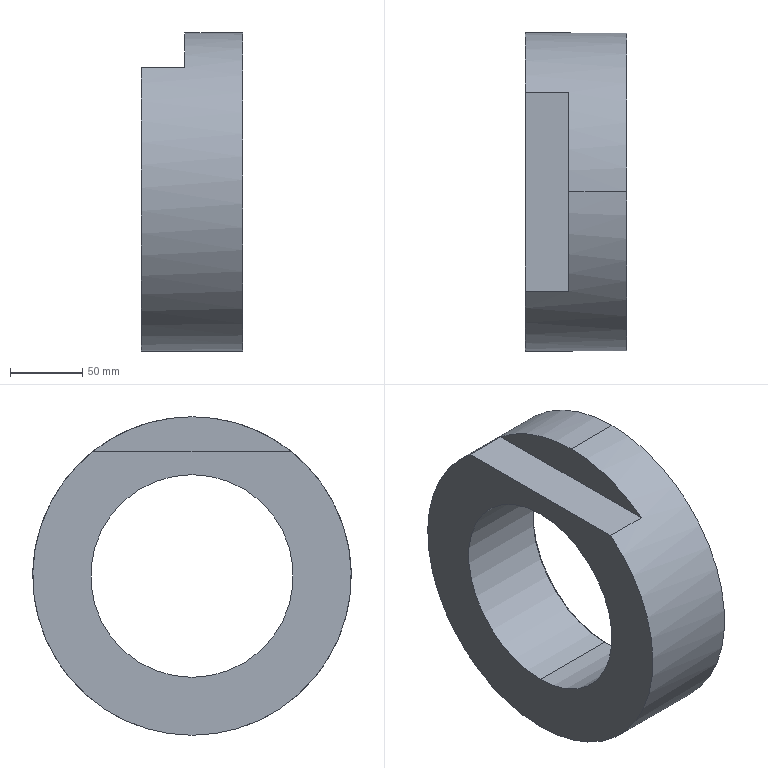Component | SolidWorks | JF21-80.1-1-3(_)-1-SOLID59-1 | 1 solid | 37 faces | box 70 x 220 x 220 mm | volume 1412143 mm3 | cylinder 18 | cone 14 | plane 5 | commonest cylinder face diameters 10.2 x12 205 x2 220 x2 140 x2
STEP:
#1=CARTESIAN_POINT('',(17.047,0.,24.37));
#2=VERTEX_POINT('',#1);
#3=CARTESIAN_POINT('',(17.047,0.,18.858));
#4=VERTEX_POINT('',#3);
#5=CARTESIAN_POINT('',(17.047,0.,21.614));
#6=DIRECTION('',(1.,0.,0.));
#7=DIRECTION('',(0.,0.,-1.));
#8=AXIS2_PLACEMENT_3D('',#5,#6,#7);
#9=CIRCLE('',#8,2.756);
#10=EDGE_CURVE('',#2,#4,#9,.T.);
#11=ORIENTED_EDGE('',*,*,#10,.F.);
#12=CARTESIAN_POINT('',(17.126,0.,24.449));
#13=VERTEX_POINT('',#12);
#14=CARTESIAN_POINT('',(17.126,0.,24.449));
#15=DIRECTION('',(-0.7071,-0.,-0.7071));
#16=VECTOR('',#15,39.37);
#17=LINE('',#14,#16);
#18=EDGE_CURVE('',#13,#2,#17,.T.);
#19=ORIENTED_EDGE('',*,*,#18,.F.);
#20=CARTESIAN_POINT('',(17.126,0.,18.78));
#21=VERTEX_POINT('',#20);
#22=CARTESIAN_POINT('',(17.126,0.,21.614));
#23=DIRECTION('',(-1.,0.,0.));
#24=DIRECTION('',(0.,0.,-1.));
#25=AXIS2_PLACEMENT_3D('',#22,#23,#24);
#26=CIRCLE('',#25,2.835);
#27=EDGE_CURVE('',#21,#13,#26,.T.);
#28=ORIENTED_EDGE('',*,*,#27,.F.);
#29=CARTESIAN_POINT('',(17.126,0.,18.78));
#30=DIRECTION('',(-0.7071,0.,0.7071));
#31=VECTOR('',#30,39.37);
#32=LINE('',#29,#31);
#33=EDGE_CURVE('',#21,#4,#32,.T.);
#34=ORIENTED_EDGE('',*,*,#33,.T.);
#35=EDGE_LOOP('',(#11,#19,#28,#34));
#36=FACE_OUTER_BOUND('',#35,.T.);
#37=CARTESIAN_POINT('',(17.126,0.,21.614));
#38=DIRECTION('',(1.,0.,0.));
#39=DIRECTION('',(0.,0.,1.));
#40=AXIS2_PLACEMENT_3D('',#37,#38,#39);
#41=CONICAL_SURFACE('',#40,2.835,0.7854);
#42=ADVANCED_FACE('',(#36),#41,.F.);
#43=CARTESIAN_POINT('',(15.974,2.898,20.142));
#44=VERTEX_POINT('',#43);
#45=CARTESIAN_POINT('',(15.974,2.898,19.74));
#46=VERTEX_POINT('',#45);
#47=CARTESIAN_POINT('',(15.974,2.898,19.941));
#48=DIRECTION('',(1.,0.,0.));
#49=DIRECTION('',(0.,0.,-1.));
#50=AXIS2_PLACEMENT_3D('',#47,#48,#49);
#51=CIRCLE('',#50,0.2008);
#52=EDGE_CURVE('',#44,#46,#51,.T.);
#53=ORIENTED_EDGE('',*,*,#52,.F.);
#54=CARTESIAN_POINT('',(17.126,2.898,20.142));
#55=VERTEX_POINT('',#54);
#56=CARTESIAN_POINT('',(17.126,2.898,20.142));
#57=DIRECTION('',(-1.,0.,0.));
#58=VECTOR('',#57,39.37);
#59=LINE('',#56,#58);
#60=EDGE_CURVE('',#55,#44,#59,.T.);
#61=ORIENTED_EDGE('',*,*,#60,.F.);
#62=CARTESIAN_POINT('',(17.126,2.898,19.74));
#63=VERTEX_POINT('',#62);
#64=CARTESIAN_POINT('',(17.126,2.898,19.941));
#65=DIRECTION('',(1.,0.,0.));
#66=DIRECTION('',(0.,0.,-1.));
#67=AXIS2_PLACEMENT_3D('',#64,#65,#66);
#68=CIRCLE('',#67,0.2008);
#69=EDGE_CURVE('',#55,#63,#68,.T.);
#70=ORIENTED_EDGE('',*,*,#69,.T.);
#71=CARTESIAN_POINT('',(17.126,2.898,19.74));
#72=DIRECTION('',(-1.,0.,0.));
#73=VECTOR('',#72,39.37);
#74=LINE('',#71,#73);
#75=EDGE_CURVE('',#63,#46,#74,.T.);
#76=ORIENTED_EDGE('',*,*,#75,.T.);
#77=EDGE_LOOP('',(#53,#61,#70,#76));
#78=FACE_OUTER_BOUND('',#77,.T.);
#79=CARTESIAN_POINT('',(17.126,2.898,19.941));
#80=DIRECTION('',(1.,0.,0.));
#81=DIRECTION('',(0.,0.,1.));
#82=AXIS2_PLACEMENT_3D('',#79,#80,#81);
#83=CYLINDRICAL_SURFACE('',#82,0.2008);
#84=ADVANCED_FACE('',(#78),#83,.F.);
#85=CARTESIAN_POINT('',(15.854,2.898,19.941));
#86=VERTEX_POINT('',#85);
#87=CARTESIAN_POINT('',(15.974,2.898,19.74));
#88=DIRECTION('',(-0.515,0.,0.8572));
#89=VECTOR('',#88,39.37);
#90=LINE('',#87,#89);
#91=EDGE_CURVE('',#46,#86,#90,.T.);
#92=ORIENTED_EDGE('',*,*,#91,.T.);
#93=CARTESIAN_POINT('',(15.974,2.898,20.142));
#94=DIRECTION('',(-0.515,-0.,-0.8572));
#95=VECTOR('',#94,39.37);
#96=LINE('',#93,#95);
#97=EDGE_CURVE('',#44,#86,#96,.T.);
#98=ORIENTED_EDGE('',*,*,#97,.F.);
#99=ORIENTED_EDGE('',*,*,#52,.T.);
#100=EDGE_LOOP('',(#92,#98,#99));
#101=FACE_OUTER_BOUND('',#100,.T.);
#102=CARTESIAN_POINT('',(15.974,2.898,19.941));
#103=DIRECTION('',(1.,0.,0.));
#104=DIRECTION('',(0.,0.,1.));
#105=AXIS2_PLACEMENT_3D('',#102,#103,#104);
#106=CONICAL_SURFACE('',#105,0.2008,1.03);
#107=ADVANCED_FACE('',(#101),#106,.F.);
#108=CARTESIAN_POINT('',(15.974,2.898,23.488));
#109=VERTEX_POINT('',#108);
#110=CARTESIAN_POINT('',(15.974,2.898,23.087));
#111=VERTEX_POINT('',#110);
#112=CARTESIAN_POINT('',(15.974,2.898,23.287));
#113=DIRECTION('',(1.,0.,0.));
#114=DIRECTION('',(0.,0.,-1.));
#115=AXIS2_PLACEMENT_3D('',#112,#113,#114);
#116=CIRCLE('',#115,0.2008);
#117=EDGE_CURVE('',#109,#111,#116,.T.);
#118=ORIENTED_EDGE('',*,*,#117,.F.);
#119=CARTESIAN_POINT('',(17.126,2.898,23.488));
#120=VERTEX_POINT('',#119);
#121=CARTESIAN_POINT('',(17.126,2.898,23.488));
#122=DIRECTION('',(-1.,0.,0.));
#123=VECTOR('',#122,39.37);
#124=LINE('',#121,#123);
#125=EDGE_CURVE('',#120,#109,#124,.T.);
#126=ORIENTED_EDGE('',*,*,#125,.F.);
#127=CARTESIAN_POINT('',(17.126,2.898,23.087));
#128=VERTEX_POINT('',#127);
#129=CARTESIAN_POINT('',(17.126,2.898,23.287));
#130=DIRECTION('',(1.,0.,0.));
#131=DIRECTION('',(0.,0.,-1.));
#132=AXIS2_PLACEMENT_3D('',#129,#130,#131);
#133=CIRCLE('',#132,0.2008);
#134=EDGE_CURVE('',#120,#128,#133,.T.);
#135=ORIENTED_EDGE('',*,*,#134,.T.);
#136=CARTESIAN_POINT('',(17.126,2.898,23.087));
#137=DIRECTION('',(-1.,0.,0.));
#138=VECTOR('',#137,39.37);
#139=LINE('',#136,#138);
#140=EDGE_CURVE('',#128,#111,#139,.T.);
#141=ORIENTED_EDGE('',*,*,#140,.T.);
#142=EDGE_LOOP('',(#118,#126,#135,#141));
#143=FACE_OUTER_BOUND('',#142,.T.);
#144=CARTESIAN_POINT('',(17.126,2.898,23.287));
#145=DIRECTION('',(1.,0.,0.));
#146=DIRECTION('',(0.,0.,1.));
#147=AXIS2_PLACEMENT_3D('',#144,#145,#146);
#148=CYLINDRICAL_SURFACE('',#147,0.2008);
#149=ADVANCED_FACE('',(#143),#148,.F.);
#150=CARTESIAN_POINT('',(15.854,2.898,23.287));
#151=VERTEX_POINT('',#150);
#152=CARTESIAN_POINT('',(15.974,2.898,23.087));
#153=DIRECTION('',(-0.515,0.,0.8572));
#154=VECTOR('',#153,39.37);
#155=LINE('',#152,#154);
#156=EDGE_CURVE('',#111,#151,#155,.T.);
#157=ORIENTED_EDGE('',*,*,#156,.T.);
#158=CARTESIAN_POINT('',(15.974,2.898,23.488));
#159=DIRECTION('',(-0.515,-0.,-0.8572));
#160=VECTOR('',#159,39.37);
#161=LINE('',#158,#160);
#162=EDGE_CURVE('',#109,#151,#161,.T.);
#163=ORIENTED_EDGE('',*,*,#162,.F.);
#164=ORIENTED_EDGE('',*,*,#117,.T.);
#165=EDGE_LOOP('',(#157,#163,#164));
#166=FACE_OUTER_BOUND('',#165,.T.);
#167=CARTESIAN_POINT('',(15.974,2.898,23.287));
#168=DIRECTION('',(1.,0.,0.));
#169=DIRECTION('',(0.,0.,1.));
#170=AXIS2_PLACEMENT_3D('',#167,#168,#169);
#171=CONICAL_SURFACE('',#170,0.2008,1.03);
#172=ADVANCED_FACE('',(#166),#171,.F.);
#173=CARTESIAN_POINT('',(15.974,0.,25.161));
#174=VERTEX_POINT('',#173);
#175=CARTESIAN_POINT('',(15.974,0.,24.76));
#176=VERTEX_POINT('',#175);
#177=CARTESIAN_POINT('',(15.974,0.,24.961));
#178=DIRECTION('',(1.,0.,0.));
#179=DIRECTION('',(0.,0.,-1.));
#180=AXIS2_PLACEMENT_3D('',#177,#178,#179);
#181=CIRCLE('',#180,0.2008);
#182=EDGE_CURVE('',#174,#176,#181,.T.);
#183=ORIENTED_EDGE('',*,*,#182,.F.);
#184=CARTESIAN_POINT('',(17.126,0.,25.161));
#185=VERTEX_POINT('',#184);
#186=CARTESIAN_POINT('',(17.126,0.,25.161));
#187=DIRECTION('',(-1.,0.,0.));
#188=VECTOR('',#187,39.37);
#189=LINE('',#186,#188);
#190=EDGE_CURVE('',#185,#174,#189,.T.);
#191=ORIENTED_EDGE('',*,*,#190,.F.);
#192=CARTESIAN_POINT('',(17.126,0.,24.76));
#193=VERTEX_POINT('',#192);
#194=CARTESIAN_POINT('',(17.126,0.,24.961));
#195=DIRECTION('',(1.,0.,0.));
#196=DIRECTION('',(0.,0.,-1.));
#197=AXIS2_PLACEMENT_3D('',#194,#195,#196);
#198=CIRCLE('',#197,0.2008);
#199=EDGE_CURVE('',#185,#193,#198,.T.);
#200=ORIENTED_EDGE('',*,*,#199,.T.);
#201=CARTESIAN_POINT('',(17.126,0.,24.76));
#202=DIRECTION('',(-1.,0.,0.));
#203=VECTOR('',#202,39.37);
#204=LINE('',#201,#203);
#205=EDGE_CURVE('',#193,#176,#204,.T.);
#206=ORIENTED_EDGE('',*,*,#205,.T.);
#207=EDGE_LOOP('',(#183,#191,#200,#206));
#208=FACE_OUTER_BOUND('',#207,.T.);
#209=CARTESIAN_POINT('',(17.126,0.,24.961));
#210=DIRECTION('',(1.,0.,0.));
#211=DIRECTION('',(0.,0.,1.));
#212=AXIS2_PLACEMENT_3D('',#209,#210,#211);
#213=CYLINDRICAL_SURFACE('',#212,0.2008);
#214=ADVANCED_FACE('',(#208),#213,.F.);
#215=CARTESIAN_POINT('',(15.854,0.,24.961));
#216=VERTEX_POINT('',#215);
#217=CARTESIAN_POINT('',(15.974,0.,24.76));
#218=DIRECTION('',(-0.515,0.,0.8572));
#219=VECTOR('',#218,39.37);
#220=LINE('',#217,#219);
#221=EDGE_CURVE('',#176,#216,#220,.T.);
#222=ORIENTED_EDGE('',*,*,#221,.T.);
#223=CARTESIAN_POINT('',(15.974,0.,25.161));
#224=DIRECTION('',(-0.515,-0.,-0.8572));
#225=VECTOR('',#224,39.37);
#226=LINE('',#223,#225);
#227=EDGE_CURVE('',#174,#216,#226,.T.);
#228=ORIENTED_EDGE('',*,*,#227,.F.);
#229=ORIENTED_EDGE('',*,*,#182,.T.);
#230=EDGE_LOOP('',(#222,#228,#229));
#231=FACE_OUTER_BOUND('',#230,.T.);
#232=CARTESIAN_POINT('',(15.974,0.,24.961));
#233=DIRECTION('',(1.,0.,0.));
#234=DIRECTION('',(0.,0.,1.));
#235=AXIS2_PLACEMENT_3D('',#232,#233,#234);
#236=CONICAL_SURFACE('',#235,0.2008,1.03);
#237=ADVANCED_FACE('',(#231),#236,.F.);
#238=CARTESIAN_POINT('',(15.974,-2.898,23.488));
#239=VERTEX_POINT('',#238);
#240=CARTESIAN_POINT('',(15.974,-2.898,23.087));
#241=VERTEX_POINT('',#240);
#242=CARTESIAN_POINT('',(15.974,-2.898,23.287));
#243=DIRECTION('',(1.,0.,0.));
#244=DIRECTION('',(0.,0.,-1.));
#245=AXIS2_PLACEMENT_3D('',#242,#243,#244);
#246=CIRCLE('',#245,0.2008);
#247=EDGE_CURVE('',#239,#241,#246,.T.);
#248=ORIENTED_EDGE('',*,*,#247,.F.);
#249=CARTESIAN_POINT('',(17.126,-2.898,23.488));
#250=VERTEX_POINT('',#249);
#251=CARTESIAN_POINT('',(17.126,-2.898,23.488));
#252=DIRECTION('',(-1.,0.,0.));
#253=VECTOR('',#252,39.37);
#254=LINE('',#251,#253);
#255=EDGE_CURVE('',#250,#239,#254,.T.);
#256=ORIENTED_EDGE('',*,*,#255,.F.);
#257=CARTESIAN_POINT('',(17.126,-2.898,23.087));
#258=VERTEX_POINT('',#257);
#259=CARTESIAN_POINT('',(17.126,-2.898,23.287));
#260=DIRECTION('',(1.,0.,0.));
#261=DIRECTION('',(0.,0.,-1.));
#262=AXIS2_PLACEMENT_3D('',#259,#260,#261);
#263=CIRCLE('',#262,0.2008);
#264=EDGE_CURVE('',#250,#258,#263,.T.);
#265=ORIENTED_EDGE('',*,*,#264,.T.);
#266=CARTESIAN_POINT('',(17.126,-2.898,23.087));
#267=DIRECTION('',(-1.,0.,0.));
#268=VECTOR('',#267,39.37);
#269=LINE('',#266,#268);
#270=EDGE_CURVE('',#258,#241,#269,.T.);
#271=ORIENTED_EDGE('',*,*,#270,.T.);
#272=EDGE_LOOP('',(#248,#256,#265,#271));
#273=FACE_OUTER_BOUND('',#272,.T.);
#274=CARTESIAN_POINT('',(17.126,-2.898,23.287));
#275=DIRECTION('',(1.,0.,0.));
#276=DIRECTION('',(0.,0.,1.));
#277=AXIS2_PLACEMENT_3D('',#274,#275,#276);
#278=CYLINDRICAL_SURFACE('',#277,0.2008);
#279=ADVANCED_FACE('',(#273),#278,.F.);
#280=CARTESIAN_POINT('',(15.854,-2.898,23.287));
#281=VERTEX_POINT('',#280);
#282=CARTESIAN_POINT('',(15.974,-2.898,23.087));
#283=DIRECTION('',(-0.515,0.,0.8572));
#284=VECTOR('',#283,39.37);
#285=LINE('',#282,#284);
#286=EDGE_CURVE('',#241,#281,#285,.T.);
#287=ORIENTED_EDGE('',*,*,#286,.T.);
#288=CARTESIAN_POINT('',(15.974,-2.898,23.488));
#289=DIRECTION('',(-0.515,-0.,-0.8572));
#290=VECTOR('',#289,39.37);
#291=LINE('',#288,#290);
#292=EDGE_CURVE('',#239,#281,#291,.T.);
#293=ORIENTED_EDGE('',*,*,#292,.F.);
#294=ORIENTED_EDGE('',*,*,#247,.T.);
#295=EDGE_LOOP('',(#287,#293,#294));
#296=FACE_OUTER_BOUND('',#295,.T.);
#297=CARTESIAN_POINT('',(15.974,-2.898,23.287));
#298=DIRECTION('',(1.,0.,0.));
#299=DIRECTION('',(0.,0.,1.));
#300=AXIS2_PLACEMENT_3D('',#297,#298,#299);
#301=CONICAL_SURFACE('',#300,0.2008,1.03);
#302=ADVANCED_FACE('',(#296),#301,.F.);
#303=CARTESIAN_POINT('',(15.974,-2.898,20.142));
#304=VERTEX_POINT('',#303);
#305=CARTESIAN_POINT('',(15.974,-2.898,19.74));
#306=VERTEX_POINT('',#305);
#307=CARTESIAN_POINT('',(15.974,-2.898,19.941));
#308=DIRECTION('',(1.,0.,0.));
#309=DIRECTION('',(0.,0.,-1.));
#310=AXIS2_PLACEMENT_3D('',#307,#308,#309);
#311=CIRCLE('',#310,0.2008);
#312=EDGE_CURVE('',#304,#306,#311,.T.);
#313=ORIENTED_EDGE('',*,*,#312,.F.);
#314=CARTESIAN_POINT('',(17.126,-2.898,20.142));
#315=VERTEX_POINT('',#314);
#316=CARTESIAN_POINT('',(17.126,-2.898,20.142));
#317=DIRECTION('',(-1.,0.,0.));
#318=VECTOR('',#317,39.37);
#319=LINE('',#316,#318);
#320=EDGE_CURVE('',#315,#304,#319,.T.);
#321=ORIENTED_EDGE('',*,*,#320,.F.);
#322=CARTESIAN_POINT('',(17.126,-2.898,19.74));
#323=VERTEX_POINT('',#322);
#324=CARTESIAN_POINT('',(17.126,-2.898,19.941));
#325=DIRECTION('',(1.,0.,0.));
#326=DIRECTION('',(0.,0.,-1.));
#327=AXIS2_PLACEMENT_3D('',#324,#325,#326);
#328=CIRCLE('',#327,0.2008);
#329=EDGE_CURVE('',#315,#323,#328,.T.);
#330=ORIENTED_EDGE('',*,*,#329,.T.);
#331=CARTESIAN_POINT('',(17.126,-2.898,19.74));
#332=DIRECTION('',(-1.,0.,0.));
#333=VECTOR('',#332,39.37);
#334=LINE('',#331,#333);
#335=EDGE_CURVE('',#323,#306,#334,.T.);
#336=ORIENTED_EDGE('',*,*,#335,.T.);
#337=EDGE_LOOP('',(#313,#321,#330,#336));
#338=FACE_OUTER_BOUND('',#337,.T.);
#339=CARTESIAN_POINT('',(17.126,-2.898,19.941));
#340=DIRECTION('',(1.,0.,0.));
#341=DIRECTION('',(0.,0.,1.));
#342=AXIS2_PLACEMENT_3D('',#339,#340,#341);
#343=CYLINDRICAL_SURFACE('',#342,0.2008);
#344=ADVANCED_FACE('',(#338),#343,.F.);
#345=CARTESIAN_POINT('',(15.854,-2.898,19.941));
#346=VERTEX_POINT('',#345);
#347=CARTESIAN_POINT('',(15.974,-2.898,19.74));
#348=DIRECTION('',(-0.515,0.,0.8572));
#349=VECTOR('',#348,39.37);
#350=LINE('',#347,#349);
#351=EDGE_CURVE('',#306,#346,#350,.T.);
#352=ORIENTED_EDGE('',*,*,#351,.T.);
#353=CARTESIAN_POINT('',(15.974,-2.898,20.142));
#354=DIRECTION('',(-0.515,-0.,-0.8572));
#355=VECTOR('',#354,39.37);
#356=LINE('',#353,#355);
#357=EDGE_CURVE('',#304,#346,#356,.T.);
#358=ORIENTED_EDGE('',*,*,#357,.F.);
#359=ORIENTED_EDGE('',*,*,#312,.T.);
#360=EDGE_LOOP('',(#352,#358,#359));
#361=FACE_OUTER_BOUND('',#360,.T.);
#362=CARTESIAN_POINT('',(15.974,-2.898,19.941));
#363=DIRECTION('',(1.,0.,0.));
#364=DIRECTION('',(0.,0.,1.));
#365=AXIS2_PLACEMENT_3D('',#362,#363,#364);
#366=CONICAL_SURFACE('',#365,0.2008,1.03);
#367=ADVANCED_FACE('',(#361),#366,.F.);
#368=CARTESIAN_POINT('',(15.974,0.,18.469));
#369=VERTEX_POINT('',#368);
#370=CARTESIAN_POINT('',(15.974,0.,18.067));
#371=VERTEX_POINT('',#370);
#372=CARTESIAN_POINT('',(15.974,0.,18.268));
#373=DIRECTION('',(1.,0.,0.));
#374=DIRECTION('',(0.,0.,-1.));
#375=AXIS2_PLACEMENT_3D('',#372,#373,#374);
#376=CIRCLE('',#375,0.2008);
#377=EDGE_CURVE('',#369,#371,#376,.T.);
#378=ORIENTED_EDGE('',*,*,#377,.F.);
#379=CARTESIAN_POINT('',(17.126,0.,18.469));
#380=VERTEX_POINT('',#379);
#381=CARTESIAN_POINT('',(17.126,0.,18.469));
#382=DIRECTION('',(-1.,0.,0.));
#383=VECTOR('',#382,39.37);
#384=LINE('',#381,#383);
#385=EDGE_CURVE('',#380,#369,#384,.T.);
#386=ORIENTED_EDGE('',*,*,#385,.F.);
#387=CARTESIAN_POINT('',(17.126,0.,18.067));
#388=VERTEX_POINT('',#387);
#389=CARTESIAN_POINT('',(17.126,0.,18.268));
#390=DIRECTION('',(1.,0.,0.));
#391=DIRECTION('',(0.,0.,-1.));
#392=AXIS2_PLACEMENT_3D('',#389,#390,#391);
#393=CIRCLE('',#392,0.2008);
#394=EDGE_CURVE('',#380,#388,#393,.T.);
#395=ORIENTED_EDGE('',*,*,#394,.T.);
#396=CARTESIAN_POINT('',(17.126,0.,18.067));
#397=DIRECTION('',(-1.,0.,0.));
#398=VECTOR('',#397,39.37);
#399=LINE('',#396,#398);
#400=EDGE_CURVE('',#388,#371,#399,.T.);
#401=ORIENTED_EDGE('',*,*,#400,.T.);
#402=EDGE_LOOP('',(#378,#386,#395,#401));
#403=FACE_OUTER_BOUND('',#402,.T.);
#404=CARTESIAN_POINT('',(17.126,0.,18.268));
#405=DIRECTION('',(1.,0.,0.));
#406=DIRECTION('',(0.,0.,1.));
#407=AXIS2_PLACEMENT_3D('',#404,#405,#406);
#408=CYLINDRICAL_SURFACE('',#407,0.2008);
#409=ADVANCED_FACE('',(#403),#408,.F.);
#410=CARTESIAN_POINT('',(15.854,-0.,18.268));
#411=VERTEX_POINT('',#410);
#412=CARTESIAN_POINT('',(15.974,0.,18.067));
#413=DIRECTION('',(-0.515,0.,0.8572));
#414=VECTOR('',#413,39.37);
#415=LINE('',#412,#414);
#416=EDGE_CURVE('',#371,#411,#415,.T.);
#417=ORIENTED_EDGE('',*,*,#416,.T.);
#418=CARTESIAN_POINT('',(15.974,0.,18.469));
#419=DIRECTION('',(-0.515,-0.,-0.8572));
#420=VECTOR('',#419,39.37);
#421=LINE('',#418,#420);
#422=EDGE_CURVE('',#369,#411,#421,.T.);
#423=ORIENTED_EDGE('',*,*,#422,.F.);
#424=ORIENTED_EDGE('',*,*,#377,.T.);
#425=EDGE_LOOP('',(#417,#423,#424));
#426=FACE_OUTER_BOUND('',#425,.T.);
#427=CARTESIAN_POINT('',(15.974,0.,18.268));
#428=DIRECTION('',(1.,0.,0.));
#429=DIRECTION('',(0.,0.,1.));
#430=AXIS2_PLACEMENT_3D('',#427,#428,#429);
#431=CONICAL_SURFACE('',#430,0.2008,1.03);
#432=ADVANCED_FACE('',(#426),#431,.F.);
#433=CARTESIAN_POINT('',(17.126,0.,25.65));
#434=VERTEX_POINT('',#433);
#435=CARTESIAN_POINT('',(17.126,0.,17.579));
#436=VERTEX_POINT('',#435);
#437=CARTESIAN_POINT('',(17.126,0.,21.614));
#438=DIRECTION('',(1.,0.,0.));
#439=DIRECTION('',(0.,0.,-1.));
#440=AXIS2_PLACEMENT_3D('',#437,#438,#439);
#441=CIRCLE('',#440,4.035);
#442=EDGE_CURVE('',#434,#436,#441,.T.);
#443=ORIENTED_EDGE('',*,*,#442,.F.);
#444=CARTESIAN_POINT('',(17.323,0.,25.65));
#445=VERTEX_POINT('',#444);
#446=CARTESIAN_POINT('',(17.126,0.,25.65));
#447=DIRECTION('',(-1.,0.,0.));
#448=VECTOR('',#447,39.37);
#449=LINE('',#446,#448);
#450=EDGE_CURVE('',#445,#434,#449,.T.);
#451=ORIENTED_EDGE('',*,*,#450,.F.);
#452=CARTESIAN_POINT('',(17.323,0.,17.579));
#453=VERTEX_POINT('',#452);
#454=CARTESIAN_POINT('',(17.323,0.,21.614));
#455=DIRECTION('',(1.,0.,0.));
#456=DIRECTION('',(0.,0.,-1.));
#457=AXIS2_PLACEMENT_3D('',#454,#455,#456);
#458=CIRCLE('',#457,4.035);
#459=EDGE_CURVE('',#445,#453,#458,.T.);
#460=ORIENTED_EDGE('',*,*,#459,.T.);
#461=CARTESIAN_POINT('',(17.126,0.,17.579));
#462=DIRECTION('',(-1.,0.,0.));
#463=VECTOR('',#462,39.37);
#464=LINE('',#461,#463);
#465=EDGE_CURVE('',#453,#436,#464,.T.);
#466=ORIENTED_EDGE('',*,*,#465,.T.);
#467=EDGE_LOOP('',(#443,#451,#460,#466));
#468=FACE_OUTER_BOUND('',#467,.T.);
#469=CARTESIAN_POINT('',(17.126,0.,21.614));
#470=DIRECTION('',(1.,0.,0.));
#471=DIRECTION('',(0.,0.,1.));
#472=AXIS2_PLACEMENT_3D('',#469,#470,#471);
#473=CYLINDRICAL_SURFACE('',#472,4.035);
#474=ADVANCED_FACE('',(#468),#473,.F.);
#475=CARTESIAN_POINT('',(15.748,0.,25.945));
#476=VERTEX_POINT('',#475);
#477=CARTESIAN_POINT('',(15.748,2.7,25.));
#478=VERTEX_POINT('',#477);
#479=CARTESIAN_POINT('',(15.748,0.,21.614));
#480=DIRECTION('',(-1.,0.,0.));
#481=DIRECTION('',(0.,0.,1.));
#482=AXIS2_PLACEMENT_3D('',#479,#480,#481);
#483=CIRCLE('',#482,4.331);
#484=EDGE_CURVE('',#476,#478,#483,.T.);
#485=ORIENTED_EDGE('',*,*,#484,.F.);
#486=CARTESIAN_POINT('',(17.323,0.,25.945));
#487=VERTEX_POINT('',#486);
#488=CARTESIAN_POINT('',(14.567,0.,25.945));
#489=DIRECTION('',(-1.,0.,0.));
#490=VECTOR('',#489,39.37);
#491=LINE('',#488,#490);
#492=EDGE_CURVE('',#487,#476,#491,.T.);
#493=ORIENTED_EDGE('',*,*,#492,.F.);
#494=CARTESIAN_POINT('',(17.323,0.,17.283));
#495=VERTEX_POINT('',#494);
#496=CARTESIAN_POINT('',(17.323,0.,21.614));
#497=DIRECTION('',(1.,0.,0.));
#498=DIRECTION('',(0.,0.,-1.));
#499=AXIS2_PLACEMENT_3D('',#496,#497,#498);
#500=CIRCLE('',#499,4.331);
#501=EDGE_CURVE('',#495,#487,#500,.T.);
#502=ORIENTED_EDGE('',*,*,#501,.F.);
#503=CARTESIAN_POINT('',(14.567,0.,17.283));
#504=VERTEX_POINT('',#503);
#505=CARTESIAN_POINT('',(14.567,0.,17.283));
#506=DIRECTION('',(-1.,0.,0.));
#507=VECTOR('',#506,39.37);
#508=LINE('',#505,#507);
#509=EDGE_CURVE('',#495,#504,#508,.T.);
#510=ORIENTED_EDGE('',*,*,#509,.T.);
#511=CARTESIAN_POINT('',(14.567,2.7,25.));
#512=VERTEX_POINT('',#511);
#513=CARTESIAN_POINT('',(14.567,0.,21.614));
#514=DIRECTION('',(1.,0.,0.));
#515=DIRECTION('',(0.,0.,-1.));
#516=AXIS2_PLACEMENT_3D('',#513,#514,#515);
#517=CIRCLE('',#516,4.331);
#518=EDGE_CURVE('',#504,#512,#517,.T.);
#519=ORIENTED_EDGE('',*,*,#518,.T.);
#520=CARTESIAN_POINT('',(15.748,2.7,25.));
#521=DIRECTION('',(-1.,0.,0.));
#522=VECTOR('',#521,39.37);
#523=LINE('',#520,#522);
#524=EDGE_CURVE('',#478,#512,#523,.T.);
#525=ORIENTED_EDGE('',*,*,#524,.F.);
#526=EDGE_LOOP('',(#485,#493,#502,#510,#519,#525));
#527=FACE_OUTER_BOUND('',#526,.T.);
#528=CARTESIAN_POINT('',(14.567,0.,21.614));
#529=DIRECTION('',(1.,0.,0.));
#530=DIRECTION('',(0.,0.,1.));
#531=AXIS2_PLACEMENT_3D('',#528,#529,#530);
#532=CYLINDRICAL_SURFACE('',#531,4.331);
#533=ADVANCED_FACE('',(#527),#532,.T.);
#534=CARTESIAN_POINT('',(14.567,0.,24.37));
#535=VERTEX_POINT('',#534);
#536=CARTESIAN_POINT('',(14.567,0.,18.858));
#537=VERTEX_POINT('',#536);
#538=CARTESIAN_POINT('',(14.567,0.,21.614));
#539=DIRECTION('',(1.,0.,0.));
#540=DIRECTION('',(0.,0.,-1.));
#541=AXIS2_PLACEMENT_3D('',#538,#539,#540);
#542=CIRCLE('',#541,2.756);
#543=EDGE_CURVE('',#535,#537,#542,.T.);
#544=ORIENTED_EDGE('',*,*,#543,.F.);
#545=CARTESIAN_POINT('',(14.567,0.,24.37));
#546=DIRECTION('',(-1.,0.,0.));
#547=VECTOR('',#546,39.37);
#548=LINE('',#545,#547);
#549=EDGE_CURVE('',#2,#535,#548,.T.);
#550=ORIENTED_EDGE('',*,*,#549,.F.);
#551=ORIENTED_EDGE('',*,*,#10,.T.);
#552=CARTESIAN_POINT('',(14.567,0.,18.858));
#553=DIRECTION('',(-1.,0.,0.));
#554=VECTOR('',#553,39.37);
#555=LINE('',#552,#554);
#556=EDGE_CURVE('',#4,#537,#555,.T.);
#557=ORIENTED_EDGE('',*,*,#556,.T.);
#558=EDGE_LOOP('',(#544,#550,#551,#557));
#559=FACE_OUTER_BOUND('',#558,.T.);
#560=CARTESIAN_POINT('',(14.567,0.,21.614));
#561=DIRECTION('',(1.,0.,0.));
#562=DIRECTION('',(0.,0.,1.));
#563=AXIS2_PLACEMENT_3D('',#560,#561,#562);
#564=CYLINDRICAL_SURFACE('',#563,2.756);
#565=ADVANCED_FACE('',(#559),#564,.F.);
#566=ORIENTED_EDGE('',*,*,#549,.T.);
#567=CARTESIAN_POINT('',(14.567,0.,21.614));
#568=DIRECTION('',(1.,0.,0.));
#569=DIRECTION('',(0.,0.,-1.));
#570=AXIS2_PLACEMENT_3D('',#567,#568,#569);
#571=CIRCLE('',#570,2.756);
#572=EDGE_CURVE('',#537,#535,#571,.T.);
#573=ORIENTED_EDGE('',*,*,#572,.F.);
#574=ORIENTED_EDGE('',*,*,#556,.F.);
#575=CARTESIAN_POINT('',(17.047,0.,21.614));
#576=DIRECTION('',(1.,0.,0.));
#577=DIRECTION('',(0.,0.,-1.));
#578=AXIS2_PLACEMENT_3D('',#575,#576,#577);
#579=CIRCLE('',#578,2.756);
#580=EDGE_CURVE('',#4,#2,#579,.T.);
#581=ORIENTED_EDGE('',*,*,#580,.T.);
#582=EDGE_LOOP('',(#566,#573,#574,#581));
#583=FACE_OUTER_BOUND('',#582,.T.);
#584=CARTESIAN_POINT('',(14.567,0.,21.614));
#585=DIRECTION('',(1.,0.,0.));
#586=DIRECTION('',(0.,0.,1.));
#587=AXIS2_PLACEMENT_3D('',#584,#585,#586);
#588=CYLINDRICAL_SURFACE('',#587,2.756);
#589=ADVANCED_FACE('',(#583),#588,.F.);
#590=ORIENTED_EDGE('',*,*,#492,.T.);
#591=CARTESIAN_POINT('',(15.748,-2.7,25.));
#592=VERTEX_POINT('',#591);
#593=CARTESIAN_POINT('',(15.748,0.,21.614));
#594=DIRECTION('',(-1.,0.,0.));
#595=DIRECTION('',(0.,0.,1.));
#596=AXIS2_PLACEMENT_3D('',#593,#594,#595);
#597=CIRCLE('',#596,4.331);
#598=EDGE_CURVE('',#592,#476,#597,.T.);
#599=ORIENTED_EDGE('',*,*,#598,.F.);
#600=CARTESIAN_POINT('',(14.567,-2.7,25.));
#601=VERTEX_POINT('',#600);
#602=CARTESIAN_POINT('',(15.748,-2.7,25.));
#603=DIRECTION('',(-1.,0.,0.));
#604=VECTOR('',#603,39.37);
#605=LINE('',#602,#604);
#606=EDGE_CURVE('',#592,#601,#605,.T.);
#607=ORIENTED_EDGE('',*,*,#606,.T.);
#608=CARTESIAN_POINT('',(14.567,0.,21.614));
#609=DIRECTION('',(1.,0.,0.));
#610=DIRECTION('',(0.,0.,-1.));
#611=AXIS2_PLACEMENT_3D('',#608,#609,#610);
#612=CIRCLE('',#611,4.331);
#613=EDGE_CURVE('',#601,#504,#612,.T.);
#614=ORIENTED_EDGE('',*,*,#613,.T.);
#615=ORIENTED_EDGE('',*,*,#509,.F.);
#616=CARTESIAN_POINT('',(17.323,0.,21.614));
#617=DIRECTION('',(1.,0.,0.));
#618=DIRECTION('',(0.,0.,-1.));
#619=AXIS2_PLACEMENT_3D('',#616,#617,#618);
#620=CIRCLE('',#619,4.331);
#621=EDGE_CURVE('',#487,#495,#620,.T.);
#622=ORIENTED_EDGE('',*,*,#621,.F.);
#623=EDGE_LOOP('',(#590,#599,#607,#614,#615,#622));
#624=FACE_OUTER_BOUND('',#623,.T.);
#625=CARTESIAN_POINT('',(14.567,0.,21.614));
#626=DIRECTION('',(1.,0.,0.));
#627=DIRECTION('',(0.,0.,1.));
#628=AXIS2_PLACEMENT_3D('',#625,#626,#627);
#629=CYLINDRICAL_SURFACE('',#628,4.331);
#630=ADVANCED_FACE('',(#624),#629,.T.);
#631=ORIENTED_EDGE('',*,*,#572,.T.);
#632=ORIENTED_EDGE('',*,*,#543,.T.);
#633=EDGE_LOOP('',(#631,#632));
#634=FACE_BOUND('',#633,.T.);
#635=ORIENTED_EDGE('',*,*,#613,.F.);
#636=CARTESIAN_POINT('',(14.567,2.7,25.));
#637=DIRECTION('',(0.,-1.,0.));
#638=VECTOR('',#637,39.37);
#639=LINE('',#636,#638);
#640=EDGE_CURVE('',#512,#601,#639,.T.);
#641=ORIENTED_EDGE('',*,*,#640,.F.);
#642=ORIENTED_EDGE('',*,*,#518,.F.);
#643=EDGE_LOOP('',(#635,#641,#642));
#644=FACE_OUTER_BOUND('',#643,.T.);
#645=CARTESIAN_POINT('',(14.567,0.,21.614));
#646=DIRECTION('',(1.,0.,0.));
#647=DIRECTION('',(0.,0.,1.));
#648=AXIS2_PLACEMENT_3D('',#645,#646,#647);
#649=PLANE('',#648);
#650=ADVANCED_FACE('',(#634,#644),#649,.F.);
#651=CARTESIAN_POINT('',(17.323,0.,21.614));
#652=DIRECTION('',(1.,0.,0.));
#653=DIRECTION('',(0.,0.,-1.));
#654=AXIS2_PLACEMENT_3D('',#651,#652,#653);
#655=CIRCLE('',#654,4.035);
#656=EDGE_CURVE('',#453,#445,#655,.T.);
#657=ORIENTED_EDGE('',*,*,#656,.F.);
#658=ORIENTED_EDGE('',*,*,#459,.F.);
#659=EDGE_LOOP('',(#657,#658));
#660=FACE_BOUND('',#659,.T.);
#661=ORIENTED_EDGE('',*,*,#501,.T.);
#662=ORIENTED_EDGE('',*,*,#621,.T.);
#663=EDGE_LOOP('',(#661,#662));
#664=FACE_OUTER_BOUND('',#663,.T.);
#665=CARTESIAN_POINT('',(17.323,0.,21.614));
#666=DIRECTION('',(1.,0.,0.));
#667=DIRECTION('',(0.,0.,1.));
#668=AXIS2_PLACEMENT_3D('',#665,#666,#667);
#669=PLANE('',#668);
#670=ADVANCED_FACE('',(#660,#664),#669,.T.);
#671=ORIENTED_EDGE('',*,*,#640,.T.);
#672=ORIENTED_EDGE('',*,*,#606,.F.);
#673=CARTESIAN_POINT('',(15.748,2.7,25.));
#674=DIRECTION('',(0.,-1.,0.));
#675=VECTOR('',#674,39.37);
#676=LINE('',#673,#675);
#677=EDGE_CURVE('',#478,#592,#676,.T.);
#678=ORIENTED_EDGE('',*,*,#677,.F.);
#679=ORIENTED_EDGE('',*,*,#524,.T.);
#680=EDGE_LOOP('',(#671,#672,#678,#679));
#681=FACE_OUTER_BOUND('',#680,.T.);
#682=CARTESIAN_POINT('',(15.748,2.7,25.));
#683=DIRECTION('',(0.,0.,-1.));
#684=DIRECTION('',(1.,0.,0.));
#685=AXIS2_PLACEMENT_3D('',#682,#683,#684);
#686=PLANE('',#685);
#687=ADVANCED_FACE('',(#681),#686,.F.);
#688=ORIENTED_EDGE('',*,*,#598,.T.);
#689=ORIENTED_EDGE('',*,*,#484,.T.);
#690=ORIENTED_EDGE('',*,*,#677,.T.);
#691=EDGE_LOOP('',(#688,#689,#690));
#692=FACE_OUTER_BOUND('',#691,.T.);
#693=CARTESIAN_POINT('',(15.748,0.,21.614));
#694=DIRECTION('',(-1.,0.,0.));
#695=DIRECTION('',(0.,0.,-1.));
#696=AXIS2_PLACEMENT_3D('',#693,#694,#695);
#697=PLANE('',#696);
#698=ADVANCED_FACE('',(#692),#697,.T.);
#699=ORIENTED_EDGE('',*,*,#27,.T.);
#700=CARTESIAN_POINT('',(17.126,0.,21.614));
#701=DIRECTION('',(-1.,0.,0.));
#702=DIRECTION('',(0.,0.,-1.));
#703=AXIS2_PLACEMENT_3D('',#700,#701,#702);
#704=CIRCLE('',#703,2.835);
#705=EDGE_CURVE('',#13,#21,#704,.T.);
#706=ORIENTED_EDGE('',*,*,#705,.T.);
#707=EDGE_LOOP('',(#699,#706));
#708=FACE_BOUND('',#707,.T.);
#709=CARTESIAN_POINT('',(17.126,2.898,19.941));
#710=DIRECTION('',(1.,0.,0.));
#711=DIRECTION('',(0.,0.,-1.));
#712=AXIS2_PLACEMENT_3D('',#709,#710,#711);
#713=CIRCLE('',#712,0.2008);
#714=EDGE_CURVE('',#63,#55,#713,.T.);
#715=ORIENTED_EDGE('',*,*,#714,.F.);
#716=ORIENTED_EDGE('',*,*,#69,.F.);
#717=EDGE_LOOP('',(#715,#716));
#718=FACE_BOUND('',#717,.T.);
#719=CARTESIAN_POINT('',(17.126,2.898,23.287));
#720=DIRECTION('',(1.,0.,0.));
#721=DIRECTION('',(0.,0.,-1.));
#722=AXIS2_PLACEMENT_3D('',#719,#720,#721);
#723=CIRCLE('',#722,0.2008);
#724=EDGE_CURVE('',#128,#120,#723,.T.);
#725=ORIENTED_EDGE('',*,*,#724,.F.);
#726=ORIENTED_EDGE('',*,*,#134,.F.);
#727=EDGE_LOOP('',(#725,#726));
#728=FACE_BOUND('',#727,.T.);
#729=CARTESIAN_POINT('',(17.126,0.,24.961));
#730=DIRECTION('',(1.,0.,0.));
#731=DIRECTION('',(0.,0.,-1.));
#732=AXIS2_PLACEMENT_3D('',#729,#730,#731);
#733=CIRCLE('',#732,0.2008);
#734=EDGE_CURVE('',#193,#185,#733,.T.);
#735=ORIENTED_EDGE('',*,*,#734,.F.);
#736=ORIENTED_EDGE('',*,*,#199,.F.);
#737=EDGE_LOOP('',(#735,#736));
#738=FACE_BOUND('',#737,.T.);
#739=CARTESIAN_POINT('',(17.126,-2.898,23.287));
#740=DIRECTION('',(1.,0.,0.));
#741=DIRECTION('',(0.,0.,-1.));
#742=AXIS2_PLACEMENT_3D('',#739,#740,#741);
#743=CIRCLE('',#742,0.2008);
#744=EDGE_CURVE('',#258,#250,#743,.T.);
#745=ORIENTED_EDGE('',*,*,#744,.F.);
#746=ORIENTED_EDGE('',*,*,#264,.F.);
#747=EDGE_LOOP('',(#745,#746));
#748=FACE_BOUND('',#747,.T.);
#749=CARTESIAN_POINT('',(17.126,-2.898,19.941));
#750=DIRECTION('',(1.,0.,0.));
#751=DIRECTION('',(0.,0.,-1.));
#752=AXIS2_PLACEMENT_3D('',#749,#750,#751);
#753=CIRCLE('',#752,0.2008);
#754=EDGE_CURVE('',#323,#315,#753,.T.);
#755=ORIENTED_EDGE('',*,*,#754,.F.);
#756=ORIENTED_EDGE('',*,*,#329,.F.);
#757=EDGE_LOOP('',(#755,#756));
#758=FACE_BOUND('',#757,.T.);
#759=CARTESIAN_POINT('',(17.126,0.,18.268));
#760=DIRECTION('',(1.,0.,0.));
#761=DIRECTION('',(0.,0.,-1.));
#762=AXIS2_PLACEMENT_3D('',#759,#760,#761);
#763=CIRCLE('',#762,0.2008);
#764=EDGE_CURVE('',#388,#380,#763,.T.);
#765=ORIENTED_EDGE('',*,*,#764,.F.);
#766=ORIENTED_EDGE('',*,*,#394,.F.);
#767=EDGE_LOOP('',(#765,#766));
#768=FACE_BOUND('',#767,.T.);
#769=CARTESIAN_POINT('',(17.126,0.,21.614));
#770=DIRECTION('',(1.,0.,0.));
#771=DIRECTION('',(0.,0.,-1.));
#772=AXIS2_PLACEMENT_3D('',#769,#770,#771);
#773=CIRCLE('',#772,4.035);
#774=EDGE_CURVE('',#436,#434,#773,.T.);
#775=ORIENTED_EDGE('',*,*,#774,.T.);
#776=ORIENTED_EDGE('',*,*,#442,.T.);
#777=EDGE_LOOP('',(#775,#776));
#778=FACE_OUTER_BOUND('',#777,.T.);
#779=CARTESIAN_POINT('',(17.126,0.,21.614));
#780=DIRECTION('',(1.,0.,0.));
#781=DIRECTION('',(0.,0.,1.));
#782=AXIS2_PLACEMENT_3D('',#779,#780,#781);
#783=PLANE('',#782);
#784=ADVANCED_FACE('',(#708,#718,#728,#738,#748,#758,#768,#778),#783,.T.);
#785=ORIENTED_EDGE('',*,*,#450,.T.);
#786=ORIENTED_EDGE('',*,*,#774,.F.);
#787=ORIENTED_EDGE('',*,*,#465,.F.);
#788=ORIENTED_EDGE('',*,*,#656,.T.);
#789=EDGE_LOOP('',(#785,#786,#787,#788));
#790=FACE_OUTER_BOUND('',#789,.T.);
#791=CARTESIAN_POINT('',(17.126,0.,21.614));
#792=DIRECTION('',(1.,0.,0.));
#793=DIRECTION('',(0.,0.,1.));
#794=AXIS2_PLACEMENT_3D('',#791,#792,#793);
#795=CYLINDRICAL_SURFACE('',#794,4.035);
#796=ADVANCED_FACE('',(#790),#795,.F.);
#797=ORIENTED_EDGE('',*,*,#422,.T.);
#798=ORIENTED_EDGE('',*,*,#416,.F.);
#799=CARTESIAN_POINT('',(15.974,0.,18.268));
#800=DIRECTION('',(1.,0.,0.));
#801=DIRECTION('',(0.,0.,-1.));
#802=AXIS2_PLACEMENT_3D('',#799,#800,#801);
#803=CIRCLE('',#802,0.2008);
#804=EDGE_CURVE('',#371,#369,#803,.T.);
#805=ORIENTED_EDGE('',*,*,#804,.T.);
#806=EDGE_LOOP('',(#797,#798,#805));
#807=FACE_OUTER_BOUND('',#806,.T.);
#808=CARTESIAN_POINT('',(15.974,0.,18.268));
#809=DIRECTION('',(1.,0.,0.));
#810=DIRECTION('',(0.,0.,1.));
#811=AXIS2_PLACEMENT_3D('',#808,#809,#810);
#812=CONICAL_SURFACE('',#811,0.2008,1.03);
#813=ADVANCED_FACE('',(#807),#812,.F.);
#814=ORIENTED_EDGE('',*,*,#385,.T.);
#815=ORIENTED_EDGE('',*,*,#804,.F.);
#816=ORIENTED_EDGE('',*,*,#400,.F.);
#817=ORIENTED_EDGE('',*,*,#764,.T.);
#818=EDGE_LOOP('',(#814,#815,#816,#817));
#819=FACE_OUTER_BOUND('',#818,.T.);
#820=CARTESIAN_POINT('',(17.126,0.,18.268));
#821=DIRECTION('',(1.,0.,0.));
#822=DIRECTION('',(0.,0.,1.));
#823=AXIS2_PLACEMENT_3D('',#820,#821,#822);
#824=CYLINDRICAL_SURFACE('',#823,0.2008);
#825=ADVANCED_FACE('',(#819),#824,.F.);
#826=ORIENTED_EDGE('',*,*,#357,.T.);
#827=ORIENTED_EDGE('',*,*,#351,.F.);
#828=CARTESIAN_POINT('',(15.974,-2.898,19.941));
#829=DIRECTION('',(1.,0.,0.));
#830=DIRECTION('',(0.,0.,-1.));
#831=AXIS2_PLACEMENT_3D('',#828,#829,#830);
#832=CIRCLE('',#831,0.2008);
#833=EDGE_CURVE('',#306,#304,#832,.T.);
#834=ORIENTED_EDGE('',*,*,#833,.T.);
#835=EDGE_LOOP('',(#826,#827,#834));
#836=FACE_OUTER_BOUND('',#835,.T.);
#837=CARTESIAN_POINT('',(15.974,-2.898,19.941));
#838=DIRECTION('',(1.,0.,0.));
#839=DIRECTION('',(0.,0.,1.));
#840=AXIS2_PLACEMENT_3D('',#837,#838,#839);
#841=CONICAL_SURFACE('',#840,0.2008,1.03);
#842=ADVANCED_FACE('',(#836),#841,.F.);
#843=ORIENTED_EDGE('',*,*,#320,.T.);
#844=ORIENTED_EDGE('',*,*,#833,.F.);
#845=ORIENTED_EDGE('',*,*,#335,.F.);
#846=ORIENTED_EDGE('',*,*,#754,.T.);
#847=EDGE_LOOP('',(#843,#844,#845,#846));
#848=FACE_OUTER_BOUND('',#847,.T.);
#849=CARTESIAN_POINT('',(17.126,-2.898,19.941));
#850=DIRECTION('',(1.,0.,0.));
#851=DIRECTION('',(0.,0.,1.));
#852=AXIS2_PLACEMENT_3D('',#849,#850,#851);
#853=CYLINDRICAL_SURFACE('',#852,0.2008);
#854=ADVANCED_FACE('',(#848),#853,.F.);
#855=ORIENTED_EDGE('',*,*,#292,.T.);
#856=ORIENTED_EDGE('',*,*,#286,.F.);
#857=CARTESIAN_POINT('',(15.974,-2.898,23.287));
#858=DIRECTION('',(1.,0.,0.));
#859=DIRECTION('',(0.,0.,-1.));
#860=AXIS2_PLACEMENT_3D('',#857,#858,#859);
#861=CIRCLE('',#860,0.2008);
#862=EDGE_CURVE('',#241,#239,#861,.T.);
#863=ORIENTED_EDGE('',*,*,#862,.T.);
#864=EDGE_LOOP('',(#855,#856,#863));
#865=FACE_OUTER_BOUND('',#864,.T.);
#866=CARTESIAN_POINT('',(15.974,-2.898,23.287));
#867=DIRECTION('',(1.,0.,0.));
#868=DIRECTION('',(0.,0.,1.));
#869=AXIS2_PLACEMENT_3D('',#866,#867,#868);
#870=CONICAL_SURFACE('',#869,0.2008,1.03);
#871=ADVANCED_FACE('',(#865),#870,.F.);
#872=ORIENTED_EDGE('',*,*,#255,.T.);
#873=ORIENTED_EDGE('',*,*,#862,.F.);
#874=ORIENTED_EDGE('',*,*,#270,.F.);
#875=ORIENTED_EDGE('',*,*,#744,.T.);
#876=EDGE_LOOP('',(#872,#873,#874,#875));
#877=FACE_OUTER_BOUND('',#876,.T.);
#878=CARTESIAN_POINT('',(17.126,-2.898,23.287));
#879=DIRECTION('',(1.,0.,0.));
#880=DIRECTION('',(0.,0.,1.));
#881=AXIS2_PLACEMENT_3D('',#878,#879,#880);
#882=CYLINDRICAL_SURFACE('',#881,0.2008);
#883=ADVANCED_FACE('',(#877),#882,.F.);
#884=ORIENTED_EDGE('',*,*,#227,.T.);
#885=ORIENTED_EDGE('',*,*,#221,.F.);
#886=CARTESIAN_POINT('',(15.974,0.,24.961));
#887=DIRECTION('',(1.,0.,0.));
#888=DIRECTION('',(0.,0.,-1.));
#889=AXIS2_PLACEMENT_3D('',#886,#887,#888);
#890=CIRCLE('',#889,0.2008);
#891=EDGE_CURVE('',#176,#174,#890,.T.);
#892=ORIENTED_EDGE('',*,*,#891,.T.);
#893=EDGE_LOOP('',(#884,#885,#892));
#894=FACE_OUTER_BOUND('',#893,.T.);
#895=CARTESIAN_POINT('',(15.974,0.,24.961));
#896=DIRECTION('',(1.,0.,0.));
#897=DIRECTION('',(0.,0.,1.));
#898=AXIS2_PLACEMENT_3D('',#895,#896,#897);
#899=CONICAL_SURFACE('',#898,0.2008,1.03);
#900=ADVANCED_FACE('',(#894),#899,.F.);
#901=ORIENTED_EDGE('',*,*,#190,.T.);
#902=ORIENTED_EDGE('',*,*,#891,.F.);
#903=ORIENTED_EDGE('',*,*,#205,.F.);
#904=ORIENTED_EDGE('',*,*,#734,.T.);
#905=EDGE_LOOP('',(#901,#902,#903,#904));
#906=FACE_OUTER_BOUND('',#905,.T.);
#907=CARTESIAN_POINT('',(17.126,0.,24.961));
#908=DIRECTION('',(1.,0.,0.));
#909=DIRECTION('',(0.,0.,1.));
#910=AXIS2_PLACEMENT_3D('',#907,#908,#909);
#911=CYLINDRICAL_SURFACE('',#910,0.2008);
#912=ADVANCED_FACE('',(#906),#911,.F.);
#913=ORIENTED_EDGE('',*,*,#162,.T.);
#914=ORIENTED_EDGE('',*,*,#156,.F.);
#915=CARTESIAN_POINT('',(15.974,2.898,23.287));
#916=DIRECTION('',(1.,0.,0.));
#917=DIRECTION('',(0.,0.,-1.));
#918=AXIS2_PLACEMENT_3D('',#915,#916,#917);
#919=CIRCLE('',#918,0.2008);
#920=EDGE_CURVE('',#111,#109,#919,.T.);
#921=ORIENTED_EDGE('',*,*,#920,.T.);
#922=EDGE_LOOP('',(#913,#914,#921));
#923=FACE_OUTER_BOUND('',#922,.T.);
#924=CARTESIAN_POINT('',(15.974,2.898,23.287));
#925=DIRECTION('',(1.,0.,0.));
#926=DIRECTION('',(0.,0.,1.));
#927=AXIS2_PLACEMENT_3D('',#924,#925,#926);
#928=CONICAL_SURFACE('',#927,0.2008,1.03);
#929=ADVANCED_FACE('',(#923),#928,.F.);
#930=ORIENTED_EDGE('',*,*,#125,.T.);
#931=ORIENTED_EDGE('',*,*,#920,.F.);
#932=ORIENTED_EDGE('',*,*,#140,.F.);
#933=ORIENTED_EDGE('',*,*,#724,.T.);
#934=EDGE_LOOP('',(#930,#931,#932,#933));
#935=FACE_OUTER_BOUND('',#934,.T.);
#936=CARTESIAN_POINT('',(17.126,2.898,23.287));
#937=DIRECTION('',(1.,0.,0.));
#938=DIRECTION('',(0.,0.,1.));
#939=AXIS2_PLACEMENT_3D('',#936,#937,#938);
#940=CYLINDRICAL_SURFACE('',#939,0.2008);
#941=ADVANCED_FACE('',(#935),#940,.F.);
#942=ORIENTED_EDGE('',*,*,#97,.T.);
#943=ORIENTED_EDGE('',*,*,#91,.F.);
#944=CARTESIAN_POINT('',(15.974,2.898,19.941));
#945=DIRECTION('',(1.,0.,0.));
#946=DIRECTION('',(0.,0.,-1.));
#947=AXIS2_PLACEMENT_3D('',#944,#945,#946);
#948=CIRCLE('',#947,0.2008);
#949=EDGE_CURVE('',#46,#44,#948,.T.);
#950=ORIENTED_EDGE('',*,*,#949,.T.);
#951=EDGE_LOOP('',(#942,#943,#950));
#952=FACE_OUTER_BOUND('',#951,.T.);
#953=CARTESIAN_POINT('',(15.974,2.898,19.941));
#954=DIRECTION('',(1.,0.,0.));
#955=DIRECTION('',(0.,0.,1.));
#956=AXIS2_PLACEMENT_3D('',#953,#954,#955);
#957=CONICAL_SURFACE('',#956,0.2008,1.03);
#958=ADVANCED_FACE('',(#952),#957,.F.);
#959=ORIENTED_EDGE('',*,*,#60,.T.);
#960=ORIENTED_EDGE('',*,*,#949,.F.);
#961=ORIENTED_EDGE('',*,*,#75,.F.);
#962=ORIENTED_EDGE('',*,*,#714,.T.);
#963=EDGE_LOOP('',(#959,#960,#961,#962));
#964=FACE_OUTER_BOUND('',#963,.T.);
#965=CARTESIAN_POINT('',(17.126,2.898,19.941));
#966=DIRECTION('',(1.,0.,0.));
#967=DIRECTION('',(0.,0.,1.));
#968=AXIS2_PLACEMENT_3D('',#965,#966,#967);
#969=CYLINDRICAL_SURFACE('',#968,0.2008);
#970=ADVANCED_FACE('',(#964),#969,.F.);
#971=ORIENTED_EDGE('',*,*,#18,.T.);
#972=ORIENTED_EDGE('',*,*,#580,.F.);
#973=ORIENTED_EDGE('',*,*,#33,.F.);
#974=ORIENTED_EDGE('',*,*,#705,.F.);
#975=EDGE_LOOP('',(#971,#972,#973,#974));
#976=FACE_OUTER_BOUND('',#975,.T.);
#977=CARTESIAN_POINT('',(17.126,0.,21.614));
#978=DIRECTION('',(1.,0.,0.));
#979=DIRECTION('',(0.,0.,1.));
#980=AXIS2_PLACEMENT_3D('',#977,#978,#979);
#981=CONICAL_SURFACE('',#980,2.835,0.7854);
#982=ADVANCED_FACE('',(#976),#981,.F.);
#983=CLOSED_SHELL('',(#42,#84,#107,#149,#172,#214,#237,#279,#302,#344,#367,#409,#432,#474,#533,#565,#589,#630,#650,#670,#687,#698,#784,#796,#813,#825,#842,#854,#871,#883,#900,#912,#929,#941,#958,#970,#982));
#984=MANIFOLD_SOLID_BREP('',#983);
#985=CARTESIAN_POINT('',(0.,0.,0.));
#986=DIRECTION('',(0.,0.,1.));
#987=DIRECTION('',(1.,0.,0.));
#988=AXIS2_PLACEMENT_3D('',#985,#986,#987);
#989=(LENGTH_UNIT()NAMED_UNIT(*)SI_UNIT($,.METRE.));
#990=LENGTH_MEASURE_WITH_UNIT(LENGTH_MEASURE(0.0254),#989);
#991=DIMENSIONAL_EXPONENTS(1.,0.,0.,0.,0.,0.,0.);
#992=(CONVERSION_BASED_UNIT('',#990)LENGTH_UNIT()NAMED_UNIT(#991));
#993=UNCERTAINTY_MEASURE_WITH_UNIT(LENGTH_MEASURE(0.00001),#992,'','');
#994=(NAMED_UNIT(*)PLANE_ANGLE_UNIT()SI_UNIT($,.RADIAN.));
#995=(NAMED_UNIT(*)SI_UNIT($,.STERADIAN.)SOLID_ANGLE_UNIT());
#996=(GEOMETRIC_REPRESENTATION_CONTEXT(3)GLOBAL_UNCERTAINTY_ASSIGNED_CONTEXT((#993))GLOBAL_UNIT_ASSIGNED_CONTEXT((#992,#994,#995))REPRESENTATION_CONTEXT('',''));
#997=ADVANCED_BREP_SHAPE_REPRESENTATION('',(#984,#988),#996);
#998=COLOUR_RGB('',0.7922,0.8196,0.9333);
#999=FILL_AREA_STYLE_COLOUR('',#998);
#1000=FILL_AREA_STYLE('',(#999));
#1001=SURFACE_STYLE_FILL_AREA(#1000);
#1002=SURFACE_SIDE_STYLE('',(#1001));
#1003=SURFACE_STYLE_USAGE(.BOTH.,#1002);
#1004=PRESENTATION_STYLE_ASSIGNMENT((#1003));
#1005=STYLED_ITEM('',(#1004),#984);
#1006=PRESENTATION_LAYER_ASSIGNMENT('','',(#1005));
#1007=(LENGTH_UNIT()NAMED_UNIT(*)SI_UNIT($,.METRE.));
#1008=LENGTH_MEASURE_WITH_UNIT(LENGTH_MEASURE(0.0254),#1007);
#1009=DIMENSIONAL_EXPONENTS(1.,0.,0.,0.,0.,0.,0.);
#1010=(CONVERSION_BASED_UNIT('',#1008)LENGTH_UNIT()NAMED_UNIT(#1009));
#1011=UNCERTAINTY_MEASURE_WITH_UNIT(LENGTH_MEASURE(0.00001),#1010,'','');
#1012=(NAMED_UNIT(*)PLANE_ANGLE_UNIT()SI_UNIT($,.RADIAN.));
#1013=(NAMED_UNIT(*)SI_UNIT($,.STERADIAN.)SOLID_ANGLE_UNIT());
#1014=(GEOMETRIC_REPRESENTATION_CONTEXT(3)GLOBAL_UNCERTAINTY_ASSIGNED_CONTEXT((#1011))GLOBAL_UNIT_ASSIGNED_CONTEXT((#1010,#1012,#1013))REPRESENTATION_CONTEXT('',''));
#1015=MECHANICAL_DESIGN_GEOMETRIC_PRESENTATION_REPRESENTATION('',(#1005),#1014);